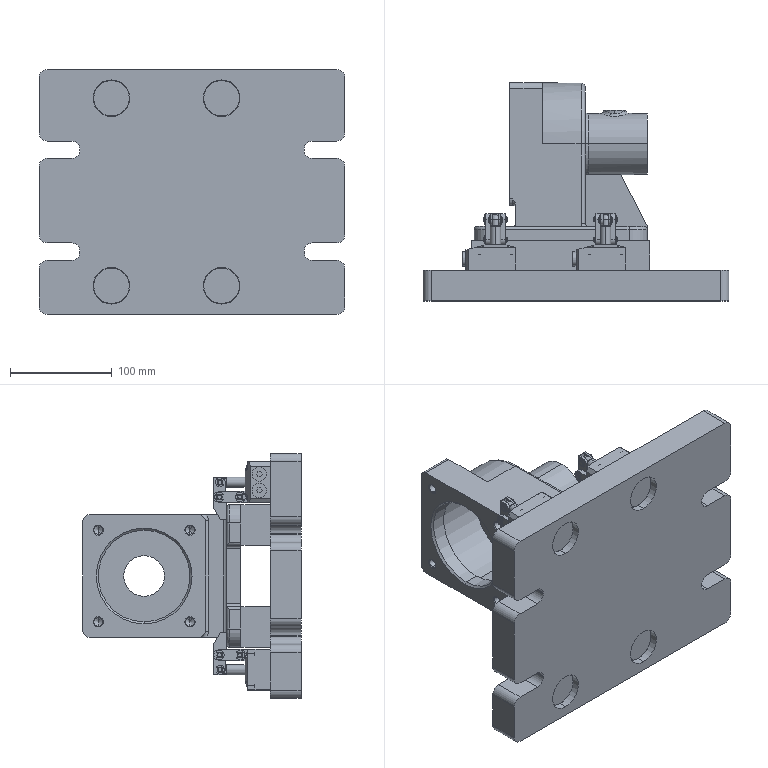Assembly | SolidWorks | mm | 98 component files | 98 solids | 2736 faces | box 300 x 214 x 240 mm | volume 3493524 mm3 | plane 1184 | cylinder 1127 | cone 265 | torus 86 | spline 66 | sphere 8 | commonest cylinder face diameters 0.8 x168 5 x148 4 x144 9 x118 3 x64 8 x48 6.4 x48 1.6 x48
Bill of materials:
10-14DiamondPin | 1 |  | Stepped pin: a plain solid cylindrical shank, a short neck of smaller diameter, then a larger faceted prismatic head whose end is cut by a conical chamfer.
Box151 | 1 |  | Bracket/housing body: a flat base plate with rounded corners, four corner holes and an open rectangular notch on one edge; an upright body with a rounded (D-shaped) end; a protruding tubular boss with a through bore; and a triangular gusset.
Box151BackingPlateDiamondPin | 1 |  | Rectangular solid bar with a row of round holes through one long face: four equally spaced larger holes on the centerline plus two smaller holes, one near each end, set off the centerline in opposite directions.
Box151BackingPlateDowelPin | 1 |  | Rectangular solid bar with a row of round holes through one long face: four equally spaced larger holes plus two smaller holes, one near each end, set off the centerline in opposite directions; the larger-hole row sits toward the opposite end compared with the similar bar.
Box151Fixture | 1 |  | Flat rectangular plate with rounded corners, four round through holes in a rectangular pattern, and two U-shaped slots cut into each of two opposite edges.
DowelPin14X30 | 1 |  | Plain solid cylinder, roughly twice as long as its diameter, with flat ends.
DowelPin8X30 | 4 |  | Plain solid cylindrical rod, roughly 3.7 times as long as its diameter, with flat ends.
hexagon socket head cap screws gb | 24 |  | Headed pin: a cylindrical head with rounded edges, a concentric circular feature on the head face, and a plain cylindrical shank with a chamfered tip.
e rings gb_GB_CONNECTING_PIECE_RINGS_HR 4 | 24 |  | Thin flat open ring (C-shape) with a wide opening on one side and three inward-projecting lobes around the inner edge, resembling an E-shaped retaining clip.
HLKA-22_-0 | 8 |  | Flat obround (slot-shaped) link plate with two round through holes, one centered in each rounded end.
HLKA-22_-1 | 4 |  | Tall rectangular bracket block with an angled cut at the top on one side, a step on the opposite side, a central slot in the lower end that forms two prongs (clevis-like), and two round through holes in the lower section.
HLKA-22_2 | 4 |  | Headed pin: a short cylindrical head with rounded edges, a long plain cylindrical shank, and a reduced flat tab at the end with a round cross hole (eye).
HLKA-22_-2 | 8 |  | Long, slender solid cylindrical pin. Each end has a narrow circumferential groove set a short distance in from the end face, and the end collars beyond the grooves are chamfered. The two ends look the same.
HLKA-22 | 4 |  | Short solid cylindrical pin with the same features as the long pin: a circumferential groove near each end and chamfered end collars. It is shorter relative to its diameter, and its grooves are wider relative to the body.
HLKA-22GL | 4 |  | Rectangular block-shaped body with a large cylindrical boss sticking out of one face. There are four through-holes near the corners. A thin tab with a single through-hole projects from one side. The edges on one end are chamfered. One side face has two circular port-like features, and an adjacent face has small recessed ring/hole features beside raised or engraved letter shapes reading 'A' and 'B'.
Part | 8 |  | Small flanged plug- or screw-like part: a short cylindrical shank with a larger-diameter, thin circular head. The head face has a hexagonal socket recess.
Mates:
1. width | Box151-1 face at (-88.619, 107.047, 70) dir (0, 0, 1) | Box151-1 face at (-88.619, 107.047, -70) dir (0, 0, -1) | Box151Fixture-1 face at (-98.619, 64.047, -120) dir (0, 0, -1) | Box151Fixture-1 face at (-98.619, 64.047, 120) dir (0, 0, 1)
2. distance | Box151-1 face at (81.381, 107.047, 70) dir (1, 0, 0) | Box151Fixture-1 face at (161.381, 64.047, 120) dir (1, 0, 0)
3. coincident | Box151-1 face at (-3.619, 107.047, 0) dir (0, 1, 0) | LeverHydraulicRod22-1/HLKA-22_-1-1 face at (-72.619, 107.047, -79) dir (0, -1, 0)
4. coincident | Box151Fixture-1 face at (51.381, 64.047, 0) dir (0, 1, 0) | LeverHydraulicRod22-1/HLKA-22GL-1 face at (-67.619, 64.047, -92) dir (0, -1, 0)
5. distance | LeverHydraulicRod22-1/HLKA-22GL-1 face at (-67.619, 64.047, -72) dir (0, 0, 1) | Box151-1 face at (-88.619, 107.047, -70) dir (0, 0, -1)
6. distance | LeverHydraulicRod22-1/HLKA-22_-1-1 face at (-62.619, 108.547, -97) dir (1, 0, 0) | Box151-1 face at (-47.619, 93.047, 0) dir (-1, 0, 0)
7. coincident | Box151-1 face at (-3.619, 107.047, 0) dir (0, 1, 0) | LeverHydraulicRod22-2/HLKA-22_-1-1 face at (35.381, 107.047, -79) dir (0, -1, 0)
8. distance | LeverHydraulicRod22-2/HLKA-22GL-1 face at (40.381, 64.047, -72) dir (0, 0, 1) | Box151-1 face at (-88.619, 107.047, -70) dir (0, 0, -1)
9. distance | LeverHydraulicRod22-2/HLKA-22_-1-1 face at (35.381, 108.547, -97) dir (-1, 0, 0) | Box151-1 face at (20.381, 188.047, 0) dir (1, 0, 0)
10. coincident | Box151-1 face at (-3.619, 107.047, 0) dir (0, 1, 0) | LeverHydraulicRod22-5/HLKA-22_-1-1 face at (45.381, 107.047, 79) dir (0, -1, 0)
11. distance | LeverHydraulicRod22-5/HLKA-22GL-1 face at (40.381, 64.047, 72) dir (0, 0, -1) | Box151-1 face at (-88.619, 107.047, 70) dir (0, 0, 1)
12. distance | LeverHydraulicRod22-5/HLKA-22_-1-1 face at (35.381, 108.547, 97) dir (-1, 0, 0) | Box151-1 face at (20.381, 188.047, 0) dir (1, 0, 0)
13. coincident | Box151-1 face at (-3.619, 107.047, 0) dir (0, 1, 0) | LeverHydraulicRod22-6/HLKA-22_-1-1 face at (-62.619, 107.047, 79) dir (0, -1, 0)
14. distance | LeverHydraulicRod22-6/HLKA-22GL-1 face at (-67.619, 64.047, 72) dir (0, 0, -1) | Box151-1 face at (-88.619, 107.047, 70) dir (0, 0, 1)
15. distance | LeverHydraulicRod22-6/HLKA-22_-1-1 face at (-62.619, 108.547, 97) dir (1, 0, 0) | Box151-1 face at (-47.619, 93.047, 0) dir (-1, 0, 0)
16. width | Box151BackingPlateDowelPin-1 face at (-91.119, 93.047, -30) dir (-1, 0, 0) | Box151BackingPlateDowelPin-1 face at (83.881, 93.047, -30) dir (1, 0, 0) | Box151-1 face at (81.381, 107.047, 70) dir (1, 0, 0) | Box151-1 face at (-88.619, 107.047, 70) dir (-1, 0, 0)
17. distance | Box151BackingPlateDowelPin-1 face at (-91.119, 93.047, -70) dir (0, 0, -1) | LeverHydraulicRod22-1/HLKA-22GL-1 face at (-67.619, 64.047, -72) dir (0, 0, 1)
18. coincident | Box151-1 face at (-3.619, 93.047, 0) dir (0, -1, 0) | Box151BackingPlateDowelPin-1 face at (-3.619, 93.047, -50) dir (0, 1, 0)
19. width | Box151BackingPlateDiamondPin-1 face at (-91.119, 93.047, 30) dir (-1, 0, 0) | Box151BackingPlateDiamondPin-1 face at (83.881, 93.047, 30) dir (1, 0, 0) | Box151-1 face at (81.381, 107.047, 70) dir (1, 0, 0) | Box151-1 face at (-88.619, 107.047, 70) dir (-1, 0, 0)
20. distance | Box151BackingPlateDiamondPin-1 face at (83.881, 93.047, 70) dir (0, 0, 1) | LeverHydraulicRod22-6/HLKA-22GL-1 face at (-67.619, 64.047, 72) dir (0, 0, -1)
21. coincident | Box151Fixture-1 face at (51.381, 64.047, 0) dir (0, 1, 0) | Box151BackingPlateDiamondPin-1 face at (-3.619, 64.047, 50) dir (0, -1, 0)
22. concentric | Box151BackingPlateDiamondPin-1 face at (-38.619, 93.047, 50) dir (0, 1, 0) r 4.5 | hexagon socket head cap screws gb-3 face at (-38.619, 78.047, 50) dir (0, 1, 0) r 0.8
23. coincident | Box151BackingPlateDiamondPin-1 face at (-43.119, 84.047, 50) dir (0, 1, 0) | hexagon socket head cap screws gb-3 face at (-38.619, 84.047, 50) dir (0, -1, 0)
24. concentric | Box151BackingPlateDiamondPin-1 face at (-73.619, 93.047, 50) dir (0, 1, 0) r 4.5 | hexagon socket head cap screws gb-4 face at (-73.619, 78.047, 50) dir (0, 1, 0) r 0.8
25. coincident | Box151BackingPlateDiamondPin-1 face at (-78.119, 84.047, 50) dir (0, 1, 0) | hexagon socket head cap screws gb-4 face at (-73.619, 84.047, 50) dir (0, -1, 0)
26. concentric | Box151BackingPlateDiamondPin-1 face at (-3.619, 93.047, 50) dir (0, 1, 0) r 4.5 | hexagon socket head cap screws gb-5 face at (-3.619, 78.047, 50) dir (0, 1, 0) r 0.8
27. coincident | Box151BackingPlateDiamondPin-1 face at (-8.119, 84.047, 50) dir (0, 1, 0) | hexagon socket head cap screws gb-5 face at (-3.619, 84.047, 50) dir (0, -1, 0)
28. concentric | Box151BackingPlateDiamondPin-1 face at (31.381, 93.047, 50) dir (0, 1, 0) r 4.5 | hexagon socket head cap screws gb-6 face at (31.381, 78.047, 50) dir (0, 1, 0) r 0.8
29. coincident | Box151BackingPlateDiamondPin-1 face at (26.881, 84.047, 50) dir (0, 1, 0) | hexagon socket head cap screws gb-6 face at (31.381, 84.047, 50) dir (0, -1, 0)
30. concentric | Box151BackingPlateDowelPin-1 face at (-38.619, 93.047, -50) dir (0, 1, 0) r 4.5 | hexagon socket head cap screws gb-7 face at (-38.619, 78.047, -50) dir (0, 1, 0) r 0.8
31. coincident | Box151BackingPlateDowelPin-1 face at (-34.119, 84.047, -50) dir (0, 1, 0) | hexagon socket head cap screws gb-7 face at (-38.619, 84.047, -50) dir (0, -1, 0)
32. concentric | Box151BackingPlateDowelPin-1 face at (-3.619, 93.047, -50) dir (0, 1, 0) r 4.5 | hexagon socket head cap screws gb-8 face at (-3.619, 78.047, -50) dir (0, 1, 0) r 0.8
33. coincident | Box151BackingPlateDowelPin-1 face at (0.8814, 84.047, -50) dir (0, 1, 0) | hexagon socket head cap screws gb-8 face at (-3.619, 84.047, -50) dir (0, -1, 0)
34. concentric | Box151BackingPlateDowelPin-1 face at (31.381, 93.047, -50) dir (0, 1, 0) r 4.5 | hexagon socket head cap screws gb-9 face at (31.381, 78.047, -50) dir (0, 1, 0) r 0.8
35. coincident | Box151BackingPlateDowelPin-1 face at (35.881, 84.047, -50) dir (0, 1, 0) | hexagon socket head cap screws gb-9 face at (31.381, 84.047, -50) dir (0, -1, 0)
36. concentric | Box151BackingPlateDowelPin-1 face at (66.381, 93.047, -50) dir (0, 1, 0) r 4.5 | hexagon socket head cap screws gb-10 face at (66.381, 78.047, -50) dir (0, 1, 0) r 0.8
37. coincident | Box151BackingPlateDowelPin-1 face at (70.881, 84.047, -50) dir (0, 1, 0) | hexagon socket head cap screws gb-10 face at (66.381, 84.047, -50) dir (0, -1, 0)
38. concentric | LeverHydraulicRod22-6/HLKA-22GL-1 face at (-83.319, 89.047, 107.7) dir (0, 1, 0) r 2.25 | hexagon socket head cap screws gb-12 face at (-83.319, 73.547, 107.7) dir (0, 1, 0) r 0.8
39. coincident | LeverHydraulicRod22-6/HLKA-22GL-1 face at (-85.569, 79.547, 107.7) dir (0, 1, 0) | hexagon socket head cap screws gb-12 face at (-83.319, 79.547, 107.7) dir (0, -1, 0)
40. concentric | LeverHydraulicRod22-6/HLKA-22GL-1 face at (-51.919, 89.047, 107.7) dir (0, 1, 0) r 2.25 | hexagon socket head cap screws gb-13 face at (-51.919, 73.547, 107.7) dir (0, 1, 0) r 0.8
41. coincident | LeverHydraulicRod22-6/HLKA-22GL-1 face at (-54.169, 79.547, 107.7) dir (0, 1, 0) | hexagon socket head cap screws gb-13 face at (-51.919, 79.547, 107.7) dir (0, -1, 0)
42. concentric | LeverHydraulicRod22-6/HLKA-22GL-1 face at (-51.919, 89.047, 76.3) dir (0, 1, 0) r 2.25 | hexagon socket head cap screws gb-14 face at (-51.919, 73.547, 76.3) dir (0, 1, 0) r 0.8
43. coincident | LeverHydraulicRod22-6/HLKA-22GL-1 face at (-54.169, 79.547, 76.3) dir (0, 1, 0) | hexagon socket head cap screws gb-14 face at (-51.919, 79.547, 76.3) dir (0, -1, 0)
44. concentric | LeverHydraulicRod22-6/HLKA-22GL-1 face at (-83.319, 89.047, 76.3) dir (0, 1, 0) r 2.25 | hexagon socket head cap screws gb-15 face at (-83.319, 73.547, 76.3) dir (0, 1, 0) r 0.8
45. coincident | LeverHydraulicRod22-6/HLKA-22GL-1 face at (-85.569, 79.547, 76.3) dir (0, 1, 0) | hexagon socket head cap screws gb-15 face at (-83.319, 79.547, 76.3) dir (0, -1, 0)
46. concentric | LeverHydraulicRod22-5/HLKA-22GL-1 face at (24.681, 89.047, 107.7) dir (0, 1, 0) r 2.25 | hexagon socket head cap screws gb-16 face at (24.681, 73.547, 107.7) dir (0, 1, 0) r 0.8
47. coincident | LeverHydraulicRod22-5/HLKA-22GL-1 face at (22.431, 79.547, 107.7) dir (0, 1, 0) | hexagon socket head cap screws gb-16 face at (24.681, 79.547, 107.7) dir (0, -1, 0)
48. concentric | LeverHydraulicRod22-5/HLKA-22GL-1 face at (56.081, 89.047, 107.7) dir (0, 1, 0) r 2.25 | hexagon socket head cap screws gb-17 face at (56.081, 73.547, 107.7) dir (0, 1, 0) r 0.8
49. coincident | LeverHydraulicRod22-5/HLKA-22GL-1 face at (53.831, 79.547, 107.7) dir (0, 1, 0) | hexagon socket head cap screws gb-17 face at (56.081, 79.547, 107.7) dir (0, -1, 0)
50. concentric | LeverHydraulicRod22-5/HLKA-22GL-1 face at (56.081, 89.047, 76.3) dir (0, 1, 0) r 2.25 | hexagon socket head cap screws gb-18 face at (56.081, 73.547, 76.3) dir (0, 1, 0) r 0.8
51. coincident | LeverHydraulicRod22-5/HLKA-22GL-1 face at (53.831, 79.547, 76.3) dir (0, 1, 0) | hexagon socket head cap screws gb-18 face at (56.081, 79.547, 76.3) dir (0, -1, 0)
52. concentric | LeverHydraulicRod22-5/HLKA-22GL-1 face at (24.681, 89.047, 76.3) dir (0, 1, 0) r 3.75 | hexagon socket head cap screws gb-19 face at (24.681, 73.547, 76.3) dir (0, 1, 0) r 0.8
53. coincident | LeverHydraulicRod22-5/HLKA-22GL-1 face at (22.431, 79.547, 76.3) dir (0, 1, 0) | hexagon socket head cap screws gb-19 face at (24.681, 79.547, 76.3) dir (0, -1, 0)
54. concentric | LeverHydraulicRod22-2/HLKA-22GL-1 face at (56.081, 89.047, -107.7) dir (0, 1, 0) r 2.25 | hexagon socket head cap screws gb-20 face at (56.081, 73.547, -107.7) dir (0, 1, 0) r 0.8
55. coincident | LeverHydraulicRod22-2/HLKA-22GL-1 face at (58.331, 79.547, -107.7) dir (0, 1, 0) | hexagon socket head cap screws gb-20 face at (56.081, 79.547, -107.7) dir (0, -1, 0)
56. concentric | LeverHydraulicRod22-2/HLKA-22GL-1 face at (56.081, 89.047, -76.3) dir (0, 1, 0) r 2.25 | hexagon socket head cap screws gb-21 face at (56.081, 73.547, -76.3) dir (0, 1, 0) r 0.8
57. coincident | LeverHydraulicRod22-2/HLKA-22GL-1 face at (58.331, 79.547, -76.3) dir (0, 1, 0) | hexagon socket head cap screws gb-21 face at (56.081, 79.547, -76.3) dir (0, -1, 0)
58. concentric | LeverHydraulicRod22-2/HLKA-22GL-1 face at (24.681, 89.047, -76.3) dir (0, 1, 0) r 2.25 | hexagon socket head cap screws gb-22 face at (24.681, 73.547, -76.3) dir (0, 1, 0) r 0.8
59. coincident | LeverHydraulicRod22-2/HLKA-22GL-1 face at (26.931, 79.547, -76.3) dir (0, 1, 0) | hexagon socket head cap screws gb-22 face at (24.681, 79.547, -76.3) dir (0, -1, 0)
60. concentric | LeverHydraulicRod22-2/HLKA-22GL-1 face at (24.681, 89.047, -107.7) dir (0, 1, 0) r 2.25 | hexagon socket head cap screws gb-23 face at (24.681, 73.547, -107.7) dir (0, 1, 0) r 0.8
61. coincident | LeverHydraulicRod22-2/HLKA-22GL-1 face at (26.931, 79.547, -107.7) dir (0, 1, 0) | hexagon socket head cap screws gb-23 face at (24.681, 79.547, -107.7) dir (0, -1, 0)
62. concentric | LeverHydraulicRod22-1/HLKA-22GL-1 face at (-83.319, 89.047, -107.7) dir (0, 1, 0) r 3.75 | hexagon socket head cap screws gb-24 face at (-83.319, 73.547, -107.7) dir (0, 1, 0) r 0.8
63. coincident | LeverHydraulicRod22-1/HLKA-22GL-1 face at (-81.069, 79.547, -107.7) dir (0, 1, 0) | hexagon socket head cap screws gb-24 face at (-83.319, 79.547, -107.7) dir (0, -1, 0)
64. concentric | LeverHydraulicRod22-1/HLKA-22GL-1 face at (-51.919, 89.047, -107.7) dir (0, 1, 0) r 2.25 | hexagon socket head cap screws gb-25 face at (-51.919, 73.547, -107.7) dir (0, 1, 0) r 0.8
65. coincident | LeverHydraulicRod22-1/HLKA-22GL-1 face at (-49.669, 79.547, -107.7) dir (0, 1, 0) | hexagon socket head cap screws gb-25 face at (-51.919, 79.547, -107.7) dir (0, -1, 0)
66. concentric | LeverHydraulicRod22-1/HLKA-22GL-1 face at (-51.919, 89.047, -76.3) dir (0, 1, 0) r 2.25 | hexagon socket head cap screws gb-26 face at (-51.919, 73.547, -76.3) dir (0, 1, 0) r 0.8
67. coincident | LeverHydraulicRod22-1/HLKA-22GL-1 face at (-49.669, 79.547, -76.3) dir (0, 1, 0) | hexagon socket head cap screws gb-26 face at (-51.919, 79.547, -76.3) dir (0, -1, 0)
68. concentric | LeverHydraulicRod22-1/HLKA-22GL-1 face at (-83.319, 89.047, -76.3) dir (0, 1, 0) r 2.25 | hexagon socket head cap screws gb-27 face at (-83.319, 73.547, -76.3) dir (0, 1, 0) r 0.8
69. coincident | LeverHydraulicRod22-1/HLKA-22GL-1 face at (-81.069, 79.547, -76.3) dir (0, 1, 0) | hexagon socket head cap screws gb-27 face at (-83.319, 79.547, -76.3) dir (0, -1, 0)
70. concentric | Box151BackingPlateDowelPin-1 face at (-83.119, 43.047, -62) dir (0, 1, 0) r 4 | DowelPin8X30-2 face at (-83.119, 84.047, -62) dir (0, -1, 0) r 4
71. coincident | Box151Fixture-1 edge at (-83.119, 64.047, 38) dir (0, 1, 0) r 4 | DowelPin8X30-3 face at (-83.119, 84.047, 38) dir (0, -1, 0) r 4
72. coincident | Box151Fixture-1 edge at (75.881, 64.047, -38) dir (0, 1, 0) r 4 | DowelPin8X30-4 face at (75.881, 84.047, -38) dir (0, -1, 0) r 4
73. coincident | Box151Fixture-1 edge at (75.881, 64.047, 62) dir (0, 1, 0) r 4 | DowelPin8X30-1 face at (75.881, 84.047, 62) dir (0, -1, 0) r 4
74. coincident | Box151Fixture-1 face at (-83.119, 54.047, -62) dir (0, 1, 0) | DowelPin8X30-2 face at (-83.119, 54.047, -62) dir (0, -1, 0)
75. coincident | Box151Fixture-1 face at (-83.119, 54.047, 38) dir (0, 1, 0) | DowelPin8X30-3 face at (-83.119, 54.047, 38) dir (0, -1, 0)
76. coincident | Box151Fixture-1 face at (75.881, 54.047, -38) dir (0, 1, 0) | DowelPin8X30-4 face at (75.881, 54.047, -38) dir (0, -1, 0)
77. coincident | Box151Fixture-1 face at (75.881, 54.047, 62) dir (0, 1, 0) | DowelPin8X30-1 edge at (75.881, 54.047, 62) dir (0, 1, 0) r 4
78. concentric | Box151-1 face at (-70.619, 107.047, -52) dir (0, 1, 0) r 7 | DowelPin14X30-1 face at (-70.619, 103.047, -52) dir (0, -1, 0) r 7
79. coincident | Box151BackingPlateDowelPin-1 face at (-70.619, 73.047, -52) dir (0, 1, 0) | DowelPin14X30-1 face at (-70.619, 73.047, -52) dir (0, -1, 0)
80. concentric | Box151BackingPlateDiamondPin-1 face at (63.381, 73.047, 52) dir (0, 1, 0) r 5 | 10-14DiamondPin-1 face at (63.381, 76.047, 52) dir (0, -1, 0) r 5
81. coincident | Box151BackingPlateDiamondPin-1 face at (-3.619, 93.047, 50) dir (0, 1, 0) | 10-14DiamondPin-1 face at (63.381, 93.047, 47.5) dir (0, -1, 0)